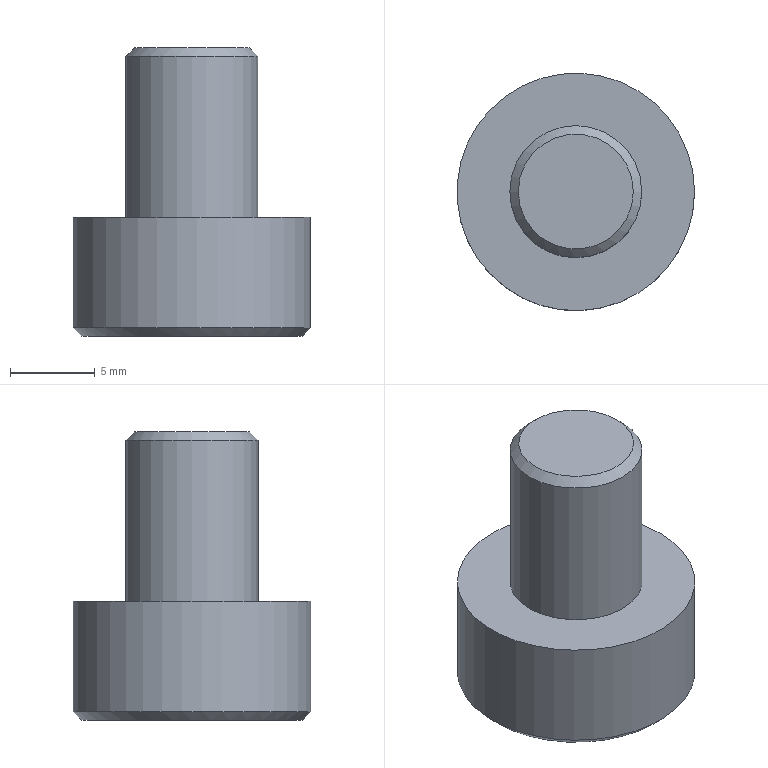Component | NX | SCREW_M8_5_2 | 1 solid | 20 faces | volume 1201 mm3 | plane 10 | cylinder 8 | cone 2 | commonest cylinder face diameters 4 x6 7.785 x1 14 x1